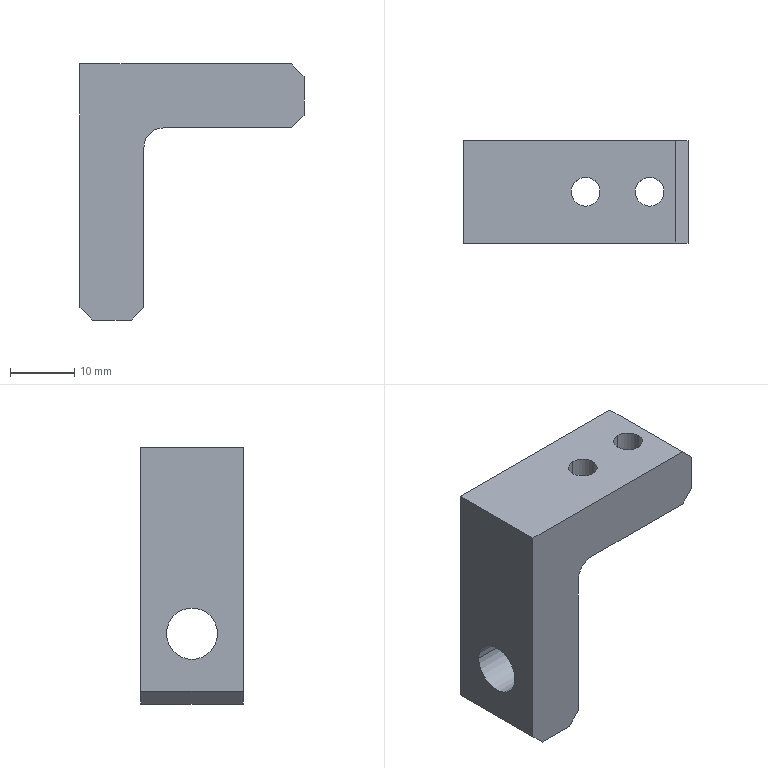Component | SolidWorks | CCDJSStopBlock01-1 | 1 solid | 25 faces | box 35 x 16 x 40 mm | volume 9180 mm3 | plane 14 | cylinder 11 | commonest cylinder face diameters 8 x6 4.5 x4 6 x1 | material 45#
build123d program:
from build123d import *

# Parameters (mm, degrees)
BOSS_EXTRUDE1_DEPTH                             = 16
FILLET1_R                                       = 3
CHAMFER1_SIZE                                   = 2
M8X1_0_TAPPED_HOLE1_D                           = 8
M4_HEX_SOCKET_HEAD_CAP_SCREW_CBORE1_D           = 4.5
M4_HEX_SOCKET_HEAD_CAP_SCREW_CBORE1_CBORE_D     = 8
M4_HEX_SOCKET_HEAD_CAP_SCREW_CBORE1_CBORE_DEPTH = 4.4


with BuildPart() as part:
    # Sketch1 → Boss-Extrude1 (new body)
    with BuildSketch(Plane.XY):
        Polygon((0, 0), (25, 0), (25, -10), (-10, -10), (-10, 30), (0, 30), align=None)
    extrude(amount=BOSS_EXTRUDE1_DEPTH)

    # Fillet1
    fillet1_edges = [part.edges().sort_by_distance(p)[0] for p in [
        (0, 0, 8),
    ]]
    fillet(fillet1_edges, radius=FILLET1_R)

    # Chamfer1
    chamfer1_edges = [part.edges().sort_by_distance(p)[0] for p in [
        (25, 0, 8),
        (25, -10, 8),
        (-10, 30, 8),
        (0, 30, 8),
    ]]
    chamfer(chamfer1_edges, length=CHAMFER1_SIZE)

    # M8x1.0 Tapped Hole1 (through all)
    with Locations(Plane.ZY.offset(10)):
        with Locations((8, 19)):
            Hole(M8X1_0_TAPPED_HOLE1_D / 2)

    # M4 Hex Socket Head Cap Screw CBORE1 (through all)
    with Locations(Plane(origin=(0, 0, 0), x_dir=(1, 0, 0), z_dir=(0, 1, 0))):
        with Locations((19, -8), (9, -8)):
            CounterBoreHole(M4_HEX_SOCKET_HEAD_CAP_SCREW_CBORE1_D / 2, M4_HEX_SOCKET_HEAD_CAP_SCREW_CBORE1_CBORE_D / 2, M4_HEX_SOCKET_HEAD_CAP_SCREW_CBORE1_CBORE_DEPTH)


solid = part.part

# Placed as in the assembly
solid = solid.moved(Location((-208, 391.564, -44.5), (-90, 0, 0)))
STEP:
#1=COLOUR_RGB('',0.7922,0.8196,0.9333);
#2=FILL_AREA_STYLE_COLOUR('',#1);
#3=FILL_AREA_STYLE('',(#2));
#4=SURFACE_STYLE_FILL_AREA(#3);
#5=SURFACE_SIDE_STYLE('',(#4));
#6=SURFACE_STYLE_USAGE(.BOTH.,#5);
#7=PRESENTATION_STYLE_ASSIGNMENT((#6));
#8=CARTESIAN_POINT('',(-7.835,15.573,-1.579));
#9=VERTEX_POINT('',#8);
#10=CARTESIAN_POINT('',(-7.835,15.888,-1.579));
#11=VERTEX_POINT('',#10);
#12=CARTESIAN_POINT('',(-7.835,15.731,-1.579));
#13=DIRECTION('',(-0.,0.,-1.));
#14=DIRECTION('',(0.,1.,0.));
#15=AXIS2_PLACEMENT_3D('',#12,#13,#14);
#16=CIRCLE('',#15,0.1575);
#17=EDGE_CURVE('',#9,#11,#16,.T.);
#18=ORIENTED_EDGE('',*,*,#17,.F.);
#19=CARTESIAN_POINT('',(-7.835,15.573,-1.752));
#20=VERTEX_POINT('',#19);
#21=CARTESIAN_POINT('',(-7.835,15.573,-1.752));
#22=DIRECTION('',(-0.,0.,-1.));
#23=VECTOR('',#22,39.37);
#24=LINE('',#21,#23);
#25=EDGE_CURVE('',#9,#20,#24,.T.);
#26=ORIENTED_EDGE('',*,*,#25,.T.);
#27=CARTESIAN_POINT('',(-7.835,15.888,-1.752));
#28=VERTEX_POINT('',#27);
#29=CARTESIAN_POINT('',(-7.835,15.731,-1.752));
#30=DIRECTION('',(-0.,0.,-1.));
#31=DIRECTION('',(0.,1.,0.));
#32=AXIS2_PLACEMENT_3D('',#29,#30,#31);
#33=CIRCLE('',#32,0.1575);
#34=EDGE_CURVE('',#20,#28,#33,.T.);
#35=ORIENTED_EDGE('',*,*,#34,.T.);
#36=CARTESIAN_POINT('',(-7.835,15.888,-1.752));
#37=DIRECTION('',(-0.,0.,-1.));
#38=VECTOR('',#37,39.37);
#39=LINE('',#36,#38);
#40=EDGE_CURVE('',#11,#28,#39,.T.);
#41=ORIENTED_EDGE('',*,*,#40,.F.);
#42=EDGE_LOOP('',(#18,#26,#35,#41));
#43=FACE_OUTER_BOUND('',#42,.T.);
#44=CARTESIAN_POINT('',(-7.835,15.731,-1.752));
#45=DIRECTION('',(-0.,0.,-1.));
#46=DIRECTION('',(0.,1.,0.));
#47=AXIS2_PLACEMENT_3D('',#44,#45,#46);
#48=CYLINDRICAL_SURFACE('',#47,0.1575);
#49=ADVANCED_FACE('',(#43),#48,.F.);
#50=CARTESIAN_POINT('',(-7.835,15.642,-1.358));
#51=VERTEX_POINT('',#50);
#52=CARTESIAN_POINT('',(-7.835,15.819,-1.358));
#53=VERTEX_POINT('',#52);
#54=CARTESIAN_POINT('',(-7.835,15.731,-1.358));
#55=DIRECTION('',(-0.,0.,-1.));
#56=DIRECTION('',(0.,1.,0.));
#57=AXIS2_PLACEMENT_3D('',#54,#55,#56);
#58=CIRCLE('',#57,0.08858);
#59=EDGE_CURVE('',#51,#53,#58,.T.);
#60=ORIENTED_EDGE('',*,*,#59,.F.);
#61=CARTESIAN_POINT('',(-7.835,15.642,-1.579));
#62=VERTEX_POINT('',#61);
#63=CARTESIAN_POINT('',(-7.835,15.642,-1.752));
#64=DIRECTION('',(-0.,0.,-1.));
#65=VECTOR('',#64,39.37);
#66=LINE('',#63,#65);
#67=EDGE_CURVE('',#51,#62,#66,.T.);
#68=ORIENTED_EDGE('',*,*,#67,.T.);
#69=CARTESIAN_POINT('',(-7.835,15.819,-1.579));
#70=VERTEX_POINT('',#69);
#71=CARTESIAN_POINT('',(-7.835,15.731,-1.579));
#72=DIRECTION('',(-0.,0.,-1.));
#73=DIRECTION('',(0.,1.,0.));
#74=AXIS2_PLACEMENT_3D('',#71,#72,#73);
#75=CIRCLE('',#74,0.08858);
#76=EDGE_CURVE('',#62,#70,#75,.T.);
#77=ORIENTED_EDGE('',*,*,#76,.T.);
#78=CARTESIAN_POINT('',(-7.835,15.819,-1.752));
#79=DIRECTION('',(-0.,0.,-1.));
#80=VECTOR('',#79,39.37);
#81=LINE('',#78,#80);
#82=EDGE_CURVE('',#53,#70,#81,.T.);
#83=ORIENTED_EDGE('',*,*,#82,.F.);
#84=EDGE_LOOP('',(#60,#68,#77,#83));
#85=FACE_OUTER_BOUND('',#84,.T.);
#86=CARTESIAN_POINT('',(-7.835,15.731,-1.752));
#87=DIRECTION('',(-0.,0.,-1.));
#88=DIRECTION('',(0.,1.,0.));
#89=AXIS2_PLACEMENT_3D('',#86,#87,#88);
#90=CYLINDRICAL_SURFACE('',#89,0.08858);
#91=ADVANCED_FACE('',(#85),#90,.F.);
#92=CARTESIAN_POINT('',(-7.441,15.573,-1.579));
#93=VERTEX_POINT('',#92);
#94=CARTESIAN_POINT('',(-7.441,15.888,-1.579));
#95=VERTEX_POINT('',#94);
#96=CARTESIAN_POINT('',(-7.441,15.731,-1.579));
#97=DIRECTION('',(-0.,0.,-1.));
#98=DIRECTION('',(0.,1.,0.));
#99=AXIS2_PLACEMENT_3D('',#96,#97,#98);
#100=CIRCLE('',#99,0.1575);
#101=EDGE_CURVE('',#93,#95,#100,.T.);
#102=ORIENTED_EDGE('',*,*,#101,.F.);
#103=CARTESIAN_POINT('',(-7.441,15.573,-1.752));
#104=VERTEX_POINT('',#103);
#105=CARTESIAN_POINT('',(-7.441,15.573,-1.752));
#106=DIRECTION('',(-0.,0.,-1.));
#107=VECTOR('',#106,39.37);
#108=LINE('',#105,#107);
#109=EDGE_CURVE('',#93,#104,#108,.T.);
#110=ORIENTED_EDGE('',*,*,#109,.T.);
#111=CARTESIAN_POINT('',(-7.441,15.888,-1.752));
#112=VERTEX_POINT('',#111);
#113=CARTESIAN_POINT('',(-7.441,15.731,-1.752));
#114=DIRECTION('',(-0.,0.,-1.));
#115=DIRECTION('',(0.,1.,0.));
#116=AXIS2_PLACEMENT_3D('',#113,#114,#115);
#117=CIRCLE('',#116,0.1575);
#118=EDGE_CURVE('',#104,#112,#117,.T.);
#119=ORIENTED_EDGE('',*,*,#118,.T.);
#120=CARTESIAN_POINT('',(-7.441,15.888,-1.752));
#121=DIRECTION('',(-0.,0.,-1.));
#122=VECTOR('',#121,39.37);
#123=LINE('',#120,#122);
#124=EDGE_CURVE('',#95,#112,#123,.T.);
#125=ORIENTED_EDGE('',*,*,#124,.F.);
#126=EDGE_LOOP('',(#102,#110,#119,#125));
#127=FACE_OUTER_BOUND('',#126,.T.);
#128=CARTESIAN_POINT('',(-7.441,15.731,-1.752));
#129=DIRECTION('',(-0.,0.,-1.));
#130=DIRECTION('',(0.,1.,0.));
#131=AXIS2_PLACEMENT_3D('',#128,#129,#130);
#132=CYLINDRICAL_SURFACE('',#131,0.1575);
#133=ADVANCED_FACE('',(#127),#132,.F.);
#134=CARTESIAN_POINT('',(-7.441,15.642,-1.358));
#135=VERTEX_POINT('',#134);
#136=CARTESIAN_POINT('',(-7.441,15.819,-1.358));
#137=VERTEX_POINT('',#136);
#138=CARTESIAN_POINT('',(-7.441,15.731,-1.358));
#139=DIRECTION('',(-0.,0.,-1.));
#140=DIRECTION('',(0.,1.,0.));
#141=AXIS2_PLACEMENT_3D('',#138,#139,#140);
#142=CIRCLE('',#141,0.08858);
#143=EDGE_CURVE('',#135,#137,#142,.T.);
#144=ORIENTED_EDGE('',*,*,#143,.F.);
#145=CARTESIAN_POINT('',(-7.441,15.642,-1.579));
#146=VERTEX_POINT('',#145);
#147=CARTESIAN_POINT('',(-7.441,15.642,-1.752));
#148=DIRECTION('',(-0.,0.,-1.));
#149=VECTOR('',#148,39.37);
#150=LINE('',#147,#149);
#151=EDGE_CURVE('',#135,#146,#150,.T.);
#152=ORIENTED_EDGE('',*,*,#151,.T.);
#153=CARTESIAN_POINT('',(-7.441,15.819,-1.579));
#154=VERTEX_POINT('',#153);
#155=CARTESIAN_POINT('',(-7.441,15.731,-1.579));
#156=DIRECTION('',(-0.,0.,-1.));
#157=DIRECTION('',(0.,1.,0.));
#158=AXIS2_PLACEMENT_3D('',#155,#156,#157);
#159=CIRCLE('',#158,0.08858);
#160=EDGE_CURVE('',#146,#154,#159,.T.);
#161=ORIENTED_EDGE('',*,*,#160,.T.);
#162=CARTESIAN_POINT('',(-7.441,15.819,-1.752));
#163=DIRECTION('',(-0.,0.,-1.));
#164=VECTOR('',#163,39.37);
#165=LINE('',#162,#164);
#166=EDGE_CURVE('',#137,#154,#165,.T.);
#167=ORIENTED_EDGE('',*,*,#166,.F.);
#168=EDGE_LOOP('',(#144,#152,#161,#167));
#169=FACE_OUTER_BOUND('',#168,.T.);
#170=CARTESIAN_POINT('',(-7.441,15.731,-1.752));
#171=DIRECTION('',(-0.,0.,-1.));
#172=DIRECTION('',(0.,1.,0.));
#173=AXIS2_PLACEMENT_3D('',#170,#171,#172);
#174=CYLINDRICAL_SURFACE('',#173,0.08858);
#175=ADVANCED_FACE('',(#169),#174,.F.);
#176=CARTESIAN_POINT('',(-8.189,15.573,-2.5));
#177=VERTEX_POINT('',#176);
#178=CARTESIAN_POINT('',(-8.189,15.888,-2.5));
#179=VERTEX_POINT('',#178);
#180=CARTESIAN_POINT('',(-8.189,15.731,-2.5));
#181=DIRECTION('',(-1.,0.,-0.));
#182=DIRECTION('',(0.,0.,1.));
#183=AXIS2_PLACEMENT_3D('',#180,#181,#182);
#184=CIRCLE('',#183,0.1575);
#185=EDGE_CURVE('',#177,#179,#184,.T.);
#186=ORIENTED_EDGE('',*,*,#185,.F.);
#187=CARTESIAN_POINT('',(-8.583,15.573,-2.5));
#188=VERTEX_POINT('',#187);
#189=CARTESIAN_POINT('',(-8.583,15.573,-2.5));
#190=DIRECTION('',(-1.,0.,0.));
#191=VECTOR('',#190,39.37);
#192=LINE('',#189,#191);
#193=EDGE_CURVE('',#177,#188,#192,.T.);
#194=ORIENTED_EDGE('',*,*,#193,.T.);
#195=CARTESIAN_POINT('',(-8.583,15.888,-2.5));
#196=VERTEX_POINT('',#195);
#197=CARTESIAN_POINT('',(-8.583,15.731,-2.5));
#198=DIRECTION('',(-1.,0.,0.));
#199=DIRECTION('',(0.,1.,0.));
#200=AXIS2_PLACEMENT_3D('',#197,#198,#199);
#201=CIRCLE('',#200,0.1575);
#202=EDGE_CURVE('',#188,#196,#201,.T.);
#203=ORIENTED_EDGE('',*,*,#202,.T.);
#204=CARTESIAN_POINT('',(-8.583,15.888,-2.5));
#205=DIRECTION('',(-1.,0.,0.));
#206=VECTOR('',#205,39.37);
#207=LINE('',#204,#206);
#208=EDGE_CURVE('',#179,#196,#207,.T.);
#209=ORIENTED_EDGE('',*,*,#208,.F.);
#210=EDGE_LOOP('',(#186,#194,#203,#209));
#211=FACE_OUTER_BOUND('',#210,.T.);
#212=CARTESIAN_POINT('',(-8.583,15.731,-2.5));
#213=DIRECTION('',(-1.,0.,0.));
#214=DIRECTION('',(0.,1.,0.));
#215=AXIS2_PLACEMENT_3D('',#212,#213,#214);
#216=CYLINDRICAL_SURFACE('',#215,0.1575);
#217=ADVANCED_FACE('',(#211),#216,.F.);
#218=CARTESIAN_POINT('',(-8.189,15.731,-2.5));
#219=DIRECTION('',(-1.,0.,-0.));
#220=DIRECTION('',(0.,0.,1.));
#221=AXIS2_PLACEMENT_3D('',#218,#219,#220);
#222=CIRCLE('',#221,0.1575);
#223=EDGE_CURVE('',#179,#177,#222,.T.);
#224=ORIENTED_EDGE('',*,*,#223,.T.);
#225=ORIENTED_EDGE('',*,*,#185,.T.);
#226=EDGE_LOOP('',(#224,#225));
#227=FACE_BOUND('',#226,.T.);
#228=CARTESIAN_POINT('',(-8.189,15.416,-1.87));
#229=VERTEX_POINT('',#228);
#230=CARTESIAN_POINT('',(-8.189,15.416,-2.854));
#231=VERTEX_POINT('',#230);
#232=CARTESIAN_POINT('',(-8.189,15.416,-2.933));
#233=DIRECTION('',(0.,0.,-1.));
#234=VECTOR('',#233,39.37);
#235=LINE('',#232,#234);
#236=EDGE_CURVE('',#229,#231,#235,.T.);
#237=ORIENTED_EDGE('',*,*,#236,.T.);
#238=CARTESIAN_POINT('',(-8.189,16.046,-2.854));
#239=VERTEX_POINT('',#238);
#240=CARTESIAN_POINT('',(-8.189,16.046,-2.854));
#241=DIRECTION('',(0.,1.,0.));
#242=VECTOR('',#241,39.37);
#243=LINE('',#240,#242);
#244=EDGE_CURVE('',#231,#239,#243,.T.);
#245=ORIENTED_EDGE('',*,*,#244,.T.);
#246=CARTESIAN_POINT('',(-8.189,16.046,-1.87));
#247=VERTEX_POINT('',#246);
#248=CARTESIAN_POINT('',(-8.189,16.046,-2.933));
#249=DIRECTION('',(0.,0.,-1.));
#250=VECTOR('',#249,39.37);
#251=LINE('',#248,#250);
#252=EDGE_CURVE('',#247,#239,#251,.T.);
#253=ORIENTED_EDGE('',*,*,#252,.F.);
#254=CARTESIAN_POINT('',(-8.189,15.416,-1.87));
#255=DIRECTION('',(-0.,-1.,-0.));
#256=VECTOR('',#255,39.37);
#257=LINE('',#254,#256);
#258=EDGE_CURVE('',#247,#229,#257,.T.);
#259=ORIENTED_EDGE('',*,*,#258,.T.);
#260=EDGE_LOOP('',(#237,#245,#253,#259));
#261=FACE_OUTER_BOUND('',#260,.T.);
#262=CARTESIAN_POINT('',(-8.189,16.046,-2.933));
#263=DIRECTION('',(-1.,0.,-0.));
#264=DIRECTION('',(-0.,-0.,1.));
#265=AXIS2_PLACEMENT_3D('',#262,#263,#264);
#266=PLANE('',#265);
#267=ADVANCED_FACE('',(#227,#261),#266,.F.);
#268=CARTESIAN_POINT('',(-8.268,15.416,-2.933));
#269=VERTEX_POINT('',#268);
#270=CARTESIAN_POINT('',(-8.504,15.416,-2.933));
#271=VERTEX_POINT('',#270);
#272=CARTESIAN_POINT('',(-8.583,15.416,-2.933));
#273=DIRECTION('',(-1.,0.,0.));
#274=VECTOR('',#273,39.37);
#275=LINE('',#272,#274);
#276=EDGE_CURVE('',#269,#271,#275,.T.);
#277=ORIENTED_EDGE('',*,*,#276,.T.);
#278=CARTESIAN_POINT('',(-8.504,16.046,-2.933));
#279=VERTEX_POINT('',#278);
#280=CARTESIAN_POINT('',(-8.504,16.046,-2.933));
#281=DIRECTION('',(0.,1.,0.));
#282=VECTOR('',#281,39.37);
#283=LINE('',#280,#282);
#284=EDGE_CURVE('',#271,#279,#283,.T.);
#285=ORIENTED_EDGE('',*,*,#284,.T.);
#286=CARTESIAN_POINT('',(-8.268,16.046,-2.933));
#287=VERTEX_POINT('',#286);
#288=CARTESIAN_POINT('',(-8.583,16.046,-2.933));
#289=DIRECTION('',(-1.,0.,0.));
#290=VECTOR('',#289,39.37);
#291=LINE('',#288,#290);
#292=EDGE_CURVE('',#287,#279,#291,.T.);
#293=ORIENTED_EDGE('',*,*,#292,.F.);
#294=CARTESIAN_POINT('',(-8.268,16.046,-2.933));
#295=DIRECTION('',(-0.,-1.,-0.));
#296=VECTOR('',#295,39.37);
#297=LINE('',#294,#296);
#298=EDGE_CURVE('',#287,#269,#297,.T.);
#299=ORIENTED_EDGE('',*,*,#298,.T.);
#300=EDGE_LOOP('',(#277,#285,#293,#299));
#301=FACE_OUTER_BOUND('',#300,.T.);
#302=CARTESIAN_POINT('',(-8.583,16.046,-2.933));
#303=DIRECTION('',(0.,-0.,1.));
#304=DIRECTION('',(-0.,-1.,-0.));
#305=AXIS2_PLACEMENT_3D('',#302,#303,#304);
#306=PLANE('',#305);
#307=ADVANCED_FACE('',(#301),#306,.F.);
#308=CARTESIAN_POINT('',(-8.583,15.731,-2.5));
#309=DIRECTION('',(-1.,0.,0.));
#310=DIRECTION('',(0.,1.,0.));
#311=AXIS2_PLACEMENT_3D('',#308,#309,#310);
#312=CIRCLE('',#311,0.1575);
#313=EDGE_CURVE('',#196,#188,#312,.T.);
#314=ORIENTED_EDGE('',*,*,#313,.F.);
#315=ORIENTED_EDGE('',*,*,#202,.F.);
#316=EDGE_LOOP('',(#314,#315));
#317=FACE_BOUND('',#316,.T.);
#318=CARTESIAN_POINT('',(-8.583,16.046,-2.854));
#319=VERTEX_POINT('',#318);
#320=CARTESIAN_POINT('',(-8.583,16.046,-1.358));
#321=VERTEX_POINT('',#320);
#322=CARTESIAN_POINT('',(-8.583,16.046,-1.358));
#323=DIRECTION('',(0.,-0.,1.));
#324=VECTOR('',#323,39.37);
#325=LINE('',#322,#324);
#326=EDGE_CURVE('',#319,#321,#325,.T.);
#327=ORIENTED_EDGE('',*,*,#326,.F.);
#328=CARTESIAN_POINT('',(-8.583,15.416,-2.854));
#329=VERTEX_POINT('',#328);
#330=CARTESIAN_POINT('',(-8.583,16.046,-2.854));
#331=DIRECTION('',(-0.,-1.,-0.));
#332=VECTOR('',#331,39.37);
#333=LINE('',#330,#332);
#334=EDGE_CURVE('',#319,#329,#333,.T.);
#335=ORIENTED_EDGE('',*,*,#334,.T.);
#336=CARTESIAN_POINT('',(-8.583,15.416,-1.358));
#337=VERTEX_POINT('',#336);
#338=CARTESIAN_POINT('',(-8.583,15.416,-1.358));
#339=DIRECTION('',(0.,-0.,1.));
#340=VECTOR('',#339,39.37);
#341=LINE('',#338,#340);
#342=EDGE_CURVE('',#329,#337,#341,.T.);
#343=ORIENTED_EDGE('',*,*,#342,.T.);
#344=CARTESIAN_POINT('',(-8.583,16.046,-1.358));
#345=DIRECTION('',(-0.,-1.,-0.));
#346=VECTOR('',#345,39.37);
#347=LINE('',#344,#346);
#348=EDGE_CURVE('',#321,#337,#347,.T.);
#349=ORIENTED_EDGE('',*,*,#348,.F.);
#350=EDGE_LOOP('',(#327,#335,#343,#349));
#351=FACE_OUTER_BOUND('',#350,.T.);
#352=CARTESIAN_POINT('',(-8.583,16.046,-1.358));
#353=DIRECTION('',(1.,-0.,-0.));
#354=DIRECTION('',(-0.,-1.,-0.));
#355=AXIS2_PLACEMENT_3D('',#352,#353,#354);
#356=PLANE('',#355);
#357=ADVANCED_FACE('',(#317,#351),#356,.F.);
#358=CARTESIAN_POINT('',(-7.835,15.731,-1.358));
#359=DIRECTION('',(-0.,0.,-1.));
#360=DIRECTION('',(0.,1.,0.));
#361=AXIS2_PLACEMENT_3D('',#358,#359,#360);
#362=CIRCLE('',#361,0.08858);
#363=EDGE_CURVE('',#53,#51,#362,.T.);
#364=ORIENTED_EDGE('',*,*,#363,.T.);
#365=ORIENTED_EDGE('',*,*,#59,.T.);
#366=EDGE_LOOP('',(#364,#365));
#367=FACE_BOUND('',#366,.T.);
#368=CARTESIAN_POINT('',(-7.441,15.731,-1.358));
#369=DIRECTION('',(-0.,0.,-1.));
#370=DIRECTION('',(0.,1.,0.));
#371=AXIS2_PLACEMENT_3D('',#368,#369,#370);
#372=CIRCLE('',#371,0.08858);
#373=EDGE_CURVE('',#137,#135,#372,.T.);
#374=ORIENTED_EDGE('',*,*,#373,.T.);
#375=ORIENTED_EDGE('',*,*,#143,.T.);
#376=EDGE_LOOP('',(#374,#375));
#377=FACE_BOUND('',#376,.T.);
#378=CARTESIAN_POINT('',(-7.283,15.416,-1.358));
#379=VERTEX_POINT('',#378);
#380=CARTESIAN_POINT('',(-7.205,15.416,-1.358));
#381=DIRECTION('',(1.,-0.,-0.));
#382=VECTOR('',#381,39.37);
#383=LINE('',#380,#382);
#384=EDGE_CURVE('',#337,#379,#383,.T.);
#385=ORIENTED_EDGE('',*,*,#384,.T.);
#386=CARTESIAN_POINT('',(-7.283,16.046,-1.358));
#387=VERTEX_POINT('',#386);
#388=CARTESIAN_POINT('',(-7.283,16.046,-1.358));
#389=DIRECTION('',(0.,1.,0.));
#390=VECTOR('',#389,39.37);
#391=LINE('',#388,#390);
#392=EDGE_CURVE('',#379,#387,#391,.T.);
#393=ORIENTED_EDGE('',*,*,#392,.T.);
#394=CARTESIAN_POINT('',(-7.205,16.046,-1.358));
#395=DIRECTION('',(1.,-0.,-0.));
#396=VECTOR('',#395,39.37);
#397=LINE('',#394,#396);
#398=EDGE_CURVE('',#321,#387,#397,.T.);
#399=ORIENTED_EDGE('',*,*,#398,.F.);
#400=ORIENTED_EDGE('',*,*,#348,.T.);
#401=EDGE_LOOP('',(#385,#393,#399,#400));
#402=FACE_OUTER_BOUND('',#401,.T.);
#403=CARTESIAN_POINT('',(-7.205,16.046,-1.358));
#404=DIRECTION('',(-0.,0.,-1.));
#405=DIRECTION('',(-1.,0.,0.));
#406=AXIS2_PLACEMENT_3D('',#403,#404,#405);
#407=PLANE('',#406);
#408=ADVANCED_FACE('',(#367,#377,#402),#407,.F.);
#409=CARTESIAN_POINT('',(-7.205,16.046,-1.437));
#410=VERTEX_POINT('',#409);
#411=CARTESIAN_POINT('',(-7.205,16.046,-1.673));
#412=VERTEX_POINT('',#411);
#413=CARTESIAN_POINT('',(-7.205,16.046,-1.752));
#414=DIRECTION('',(-0.,0.,-1.));
#415=VECTOR('',#414,39.37);
#416=LINE('',#413,#415);
#417=EDGE_CURVE('',#410,#412,#416,.T.);
#418=ORIENTED_EDGE('',*,*,#417,.F.);
#419=CARTESIAN_POINT('',(-7.205,15.416,-1.437));
#420=VERTEX_POINT('',#419);
#421=CARTESIAN_POINT('',(-7.205,16.046,-1.437));
#422=DIRECTION('',(-0.,-1.,-0.));
#423=VECTOR('',#422,39.37);
#424=LINE('',#421,#423);
#425=EDGE_CURVE('',#410,#420,#424,.T.);
#426=ORIENTED_EDGE('',*,*,#425,.T.);
#427=CARTESIAN_POINT('',(-7.205,15.416,-1.673));
#428=VERTEX_POINT('',#427);
#429=CARTESIAN_POINT('',(-7.205,15.416,-1.752));
#430=DIRECTION('',(-0.,0.,-1.));
#431=VECTOR('',#430,39.37);
#432=LINE('',#429,#431);
#433=EDGE_CURVE('',#420,#428,#432,.T.);
#434=ORIENTED_EDGE('',*,*,#433,.T.);
#435=CARTESIAN_POINT('',(-7.205,16.046,-1.673));
#436=DIRECTION('',(0.,1.,0.));
#437=VECTOR('',#436,39.37);
#438=LINE('',#435,#437);
#439=EDGE_CURVE('',#428,#412,#438,.T.);
#440=ORIENTED_EDGE('',*,*,#439,.T.);
#441=EDGE_LOOP('',(#418,#426,#434,#440));
#442=FACE_OUTER_BOUND('',#441,.T.);
#443=CARTESIAN_POINT('',(-7.205,16.046,-1.752));
#444=DIRECTION('',(-1.,0.,0.));
#445=DIRECTION('',(0.,1.,0.));
#446=AXIS2_PLACEMENT_3D('',#443,#444,#445);
#447=PLANE('',#446);
#448=ADVANCED_FACE('',(#442),#447,.F.);
#449=CARTESIAN_POINT('',(-7.835,15.731,-1.752));
#450=DIRECTION('',(-0.,0.,-1.));
#451=DIRECTION('',(0.,1.,0.));
#452=AXIS2_PLACEMENT_3D('',#449,#450,#451);
#453=CIRCLE('',#452,0.1575);
#454=EDGE_CURVE('',#28,#20,#453,.T.);
#455=ORIENTED_EDGE('',*,*,#454,.F.);
#456=ORIENTED_EDGE('',*,*,#34,.F.);
#457=EDGE_LOOP('',(#455,#456));
#458=FACE_BOUND('',#457,.T.);
#459=CARTESIAN_POINT('',(-7.283,16.046,-1.752));
#460=VERTEX_POINT('',#459);
#461=CARTESIAN_POINT('',(-7.283,15.731,-1.752));
#462=VERTEX_POINT('',#461);
#463=CARTESIAN_POINT('',(-7.283,16.046,-1.752));
#464=DIRECTION('',(-0.,-1.,-0.));
#465=VECTOR('',#464,39.37);
#466=LINE('',#463,#465);
#467=EDGE_CURVE('',#460,#462,#466,.T.);
#468=ORIENTED_EDGE('',*,*,#467,.T.);
#469=CARTESIAN_POINT('',(-7.441,15.731,-1.752));
#470=DIRECTION('',(-0.,0.,-1.));
#471=DIRECTION('',(0.,1.,0.));
#472=AXIS2_PLACEMENT_3D('',#469,#470,#471);
#473=CIRCLE('',#472,0.1575);
#474=EDGE_CURVE('',#112,#462,#473,.T.);
#475=ORIENTED_EDGE('',*,*,#474,.F.);
#476=ORIENTED_EDGE('',*,*,#118,.F.);
#477=CARTESIAN_POINT('',(-7.441,15.731,-1.752));
#478=DIRECTION('',(-0.,0.,-1.));
#479=DIRECTION('',(0.,1.,0.));
#480=AXIS2_PLACEMENT_3D('',#477,#478,#479);
#481=CIRCLE('',#480,0.1575);
#482=EDGE_CURVE('',#462,#104,#481,.T.);
#483=ORIENTED_EDGE('',*,*,#482,.F.);
#484=CARTESIAN_POINT('',(-7.283,15.416,-1.752));
#485=VERTEX_POINT('',#484);
#486=CARTESIAN_POINT('',(-7.283,16.046,-1.752));
#487=DIRECTION('',(-0.,-1.,-0.));
#488=VECTOR('',#487,39.37);
#489=LINE('',#486,#488);
#490=EDGE_CURVE('',#462,#485,#489,.T.);
#491=ORIENTED_EDGE('',*,*,#490,.T.);
#492=CARTESIAN_POINT('',(-8.071,15.416,-1.752));
#493=VERTEX_POINT('',#492);
#494=CARTESIAN_POINT('',(-8.189,15.416,-1.752));
#495=DIRECTION('',(-1.,0.,0.));
#496=VECTOR('',#495,39.37);
#497=LINE('',#494,#496);
#498=EDGE_CURVE('',#485,#493,#497,.T.);
#499=ORIENTED_EDGE('',*,*,#498,.T.);
#500=CARTESIAN_POINT('',(-8.071,16.046,-1.752));
#501=VERTEX_POINT('',#500);
#502=CARTESIAN_POINT('',(-8.071,16.046,-1.752));
#503=DIRECTION('',(0.,1.,0.));
#504=VECTOR('',#503,39.37);
#505=LINE('',#502,#504);
#506=EDGE_CURVE('',#493,#501,#505,.T.);
#507=ORIENTED_EDGE('',*,*,#506,.T.);
#508=CARTESIAN_POINT('',(-8.189,16.046,-1.752));
#509=DIRECTION('',(-1.,0.,0.));
#510=VECTOR('',#509,39.37);
#511=LINE('',#508,#510);
#512=EDGE_CURVE('',#460,#501,#511,.T.);
#513=ORIENTED_EDGE('',*,*,#512,.F.);
#514=EDGE_LOOP('',(#468,#475,#476,#483,#491,#499,#507,#513));
#515=FACE_OUTER_BOUND('',#514,.T.);
#516=CARTESIAN_POINT('',(-8.189,16.046,-1.752));
#517=DIRECTION('',(0.,-0.,1.));
#518=DIRECTION('',(-0.,-1.,-0.));
#519=AXIS2_PLACEMENT_3D('',#516,#517,#518);
#520=PLANE('',#519);
#521=ADVANCED_FACE('',(#458,#515),#520,.F.);
#522=ORIENTED_EDGE('',*,*,#398,.T.);
#523=CARTESIAN_POINT('',(-7.539,16.046,-1.102));
#524=DIRECTION('',(0.7071,-0.,-0.7071));
#525=VECTOR('',#524,39.37);
#526=LINE('',#523,#525);
#527=EDGE_CURVE('',#387,#410,#526,.T.);
#528=ORIENTED_EDGE('',*,*,#527,.T.);
#529=ORIENTED_EDGE('',*,*,#417,.T.);
#530=CARTESIAN_POINT('',(-7.736,16.046,-2.205));
#531=DIRECTION('',(-0.7071,0.,-0.7071));
#532=VECTOR('',#531,39.37);
#533=LINE('',#530,#532);
#534=EDGE_CURVE('',#412,#460,#533,.T.);
#535=ORIENTED_EDGE('',*,*,#534,.T.);
#536=ORIENTED_EDGE('',*,*,#512,.T.);
#537=CARTESIAN_POINT('',(-8.071,16.046,-1.87));
#538=DIRECTION('',(-0.,-1.,-0.));
#539=DIRECTION('',(1.,0.,0.));
#540=AXIS2_PLACEMENT_3D('',#537,#538,#539);
#541=CIRCLE('',#540,0.1181);
#542=EDGE_CURVE('',#501,#247,#541,.T.);
#543=ORIENTED_EDGE('',*,*,#542,.T.);
#544=ORIENTED_EDGE('',*,*,#252,.T.);
#545=CARTESIAN_POINT('',(-7.638,16.046,-2.303));
#546=DIRECTION('',(-0.7071,0.,-0.7071));
#547=VECTOR('',#546,39.37);
#548=LINE('',#545,#547);
#549=EDGE_CURVE('',#239,#287,#548,.T.);
#550=ORIENTED_EDGE('',*,*,#549,.T.);
#551=ORIENTED_EDGE('',*,*,#292,.T.);
#552=CARTESIAN_POINT('',(-8.937,16.046,-2.5));
#553=DIRECTION('',(-0.7071,0.,0.7071));
#554=VECTOR('',#553,39.37);
#555=LINE('',#552,#554);
#556=EDGE_CURVE('',#279,#319,#555,.T.);
#557=ORIENTED_EDGE('',*,*,#556,.T.);
#558=ORIENTED_EDGE('',*,*,#326,.T.);
#559=EDGE_LOOP('',(#522,#528,#529,#535,#536,#543,#544,#550,#551,#557,#558));
#560=FACE_OUTER_BOUND('',#559,.T.);
#561=CARTESIAN_POINT('',(-8.189,16.046,-1.752));
#562=DIRECTION('',(0.,1.,0.));
#563=DIRECTION('',(1.,-0.,-0.));
#564=AXIS2_PLACEMENT_3D('',#561,#562,#563);
#565=PLANE('',#564);
#566=ADVANCED_FACE('',(#560),#565,.T.);
#567=ORIENTED_EDGE('',*,*,#433,.F.);
#568=CARTESIAN_POINT('',(-7.205,15.416,-1.437));
#569=DIRECTION('',(-0.7071,0.,0.7071));
#570=VECTOR('',#569,39.37);
#571=LINE('',#568,#570);
#572=EDGE_CURVE('',#420,#379,#571,.T.);
#573=ORIENTED_EDGE('',*,*,#572,.T.);
#574=ORIENTED_EDGE('',*,*,#384,.F.);
#575=ORIENTED_EDGE('',*,*,#342,.F.);
#576=CARTESIAN_POINT('',(-8.583,15.416,-2.854));
#577=DIRECTION('',(0.7071,-0.,-0.7071));
#578=VECTOR('',#577,39.37);
#579=LINE('',#576,#578);
#580=EDGE_CURVE('',#329,#271,#579,.T.);
#581=ORIENTED_EDGE('',*,*,#580,.T.);
#582=ORIENTED_EDGE('',*,*,#276,.F.);
#583=CARTESIAN_POINT('',(-8.268,15.416,-2.933));
#584=DIRECTION('',(0.7071,-0.,0.7071));
#585=VECTOR('',#584,39.37);
#586=LINE('',#583,#585);
#587=EDGE_CURVE('',#269,#231,#586,.T.);
#588=ORIENTED_EDGE('',*,*,#587,.T.);
#589=ORIENTED_EDGE('',*,*,#236,.F.);
#590=CARTESIAN_POINT('',(-8.071,15.416,-1.87));
#591=DIRECTION('',(0.,1.,0.));
#592=DIRECTION('',(1.,0.,0.));
#593=AXIS2_PLACEMENT_3D('',#590,#591,#592);
#594=CIRCLE('',#593,0.1181);
#595=EDGE_CURVE('',#229,#493,#594,.T.);
#596=ORIENTED_EDGE('',*,*,#595,.T.);
#597=ORIENTED_EDGE('',*,*,#498,.F.);
#598=CARTESIAN_POINT('',(-7.283,15.416,-1.752));
#599=DIRECTION('',(0.7071,-0.,0.7071));
#600=VECTOR('',#599,39.37);
#601=LINE('',#598,#600);
#602=EDGE_CURVE('',#485,#428,#601,.T.);
#603=ORIENTED_EDGE('',*,*,#602,.T.);
#604=EDGE_LOOP('',(#567,#573,#574,#575,#581,#582,#588,#589,#596,#597,#603));
#605=FACE_OUTER_BOUND('',#604,.T.);
#606=CARTESIAN_POINT('',(-8.189,15.416,-1.752));
#607=DIRECTION('',(0.,1.,0.));
#608=DIRECTION('',(1.,-0.,-0.));
#609=AXIS2_PLACEMENT_3D('',#606,#607,#608);
#610=PLANE('',#609);
#611=ADVANCED_FACE('',(#605),#610,.F.);
#612=ORIENTED_EDGE('',*,*,#542,.F.);
#613=ORIENTED_EDGE('',*,*,#506,.F.);
#614=ORIENTED_EDGE('',*,*,#595,.F.);
#615=ORIENTED_EDGE('',*,*,#258,.F.);
#616=EDGE_LOOP('',(#612,#613,#614,#615));
#617=FACE_OUTER_BOUND('',#616,.T.);
#618=CARTESIAN_POINT('',(-8.071,16.046,-1.87));
#619=DIRECTION('',(0.,1.,0.));
#620=DIRECTION('',(1.,0.,0.));
#621=AXIS2_PLACEMENT_3D('',#618,#619,#620);
#622=CYLINDRICAL_SURFACE('',#621,0.1181);
#623=ADVANCED_FACE('',(#617),#622,.F.);
#624=ORIENTED_EDGE('',*,*,#527,.F.);
#625=ORIENTED_EDGE('',*,*,#392,.F.);
#626=ORIENTED_EDGE('',*,*,#572,.F.);
#627=ORIENTED_EDGE('',*,*,#425,.F.);
#628=EDGE_LOOP('',(#624,#625,#626,#627));
#629=FACE_OUTER_BOUND('',#628,.T.);
#630=CARTESIAN_POINT('',(-7.205,16.046,-1.437));
#631=DIRECTION('',(-0.7071,0.,-0.7071));
#632=DIRECTION('',(-0.,-1.,-0.));
#633=AXIS2_PLACEMENT_3D('',#630,#631,#632);
#634=PLANE('',#633);
#635=ADVANCED_FACE('',(#629),#634,.F.);
#636=ORIENTED_EDGE('',*,*,#534,.F.);
#637=ORIENTED_EDGE('',*,*,#439,.F.);
#638=ORIENTED_EDGE('',*,*,#602,.F.);
#639=ORIENTED_EDGE('',*,*,#490,.F.);
#640=ORIENTED_EDGE('',*,*,#467,.F.);
#641=EDGE_LOOP('',(#636,#637,#638,#639,#640));
#642=FACE_OUTER_BOUND('',#641,.T.);
#643=CARTESIAN_POINT('',(-7.283,16.046,-1.752));
#644=DIRECTION('',(-0.7071,0.,0.7071));
#645=DIRECTION('',(-0.,-1.,-0.));
#646=AXIS2_PLACEMENT_3D('',#643,#644,#645);
#647=PLANE('',#646);
#648=ADVANCED_FACE('',(#642),#647,.F.);
#649=ORIENTED_EDGE('',*,*,#556,.F.);
#650=ORIENTED_EDGE('',*,*,#284,.F.);
#651=ORIENTED_EDGE('',*,*,#580,.F.);
#652=ORIENTED_EDGE('',*,*,#334,.F.);
#653=EDGE_LOOP('',(#649,#650,#651,#652));
#654=FACE_OUTER_BOUND('',#653,.T.);
#655=CARTESIAN_POINT('',(-8.583,16.046,-2.854));
#656=DIRECTION('',(0.7071,-0.,0.7071));
#657=DIRECTION('',(-0.,-1.,-0.));
#658=AXIS2_PLACEMENT_3D('',#655,#656,#657);
#659=PLANE('',#658);
#660=ADVANCED_FACE('',(#654),#659,.F.);
#661=ORIENTED_EDGE('',*,*,#549,.F.);
#662=ORIENTED_EDGE('',*,*,#244,.F.);
#663=ORIENTED_EDGE('',*,*,#587,.F.);
#664=ORIENTED_EDGE('',*,*,#298,.F.);
#665=EDGE_LOOP('',(#661,#662,#663,#664));
#666=FACE_OUTER_BOUND('',#665,.T.);
#667=CARTESIAN_POINT('',(-8.268,16.046,-2.933));
#668=DIRECTION('',(-0.7071,0.,0.7071));
#669=DIRECTION('',(-0.,-1.,-0.));
#670=AXIS2_PLACEMENT_3D('',#667,#668,#669);
#671=PLANE('',#670);
#672=ADVANCED_FACE('',(#666),#671,.F.);
#673=ORIENTED_EDGE('',*,*,#193,.F.);
#674=ORIENTED_EDGE('',*,*,#223,.F.);
#675=ORIENTED_EDGE('',*,*,#208,.T.);
#676=ORIENTED_EDGE('',*,*,#313,.T.);
#677=EDGE_LOOP('',(#673,#674,#675,#676));
#678=FACE_OUTER_BOUND('',#677,.T.);
#679=CARTESIAN_POINT('',(-8.583,15.731,-2.5));
#680=DIRECTION('',(-1.,0.,0.));
#681=DIRECTION('',(0.,1.,0.));
#682=AXIS2_PLACEMENT_3D('',#679,#680,#681);
#683=CYLINDRICAL_SURFACE('',#682,0.1575);
#684=ADVANCED_FACE('',(#678),#683,.F.);
#685=ORIENTED_EDGE('',*,*,#151,.F.);
#686=ORIENTED_EDGE('',*,*,#373,.F.);
#687=ORIENTED_EDGE('',*,*,#166,.T.);
#688=CARTESIAN_POINT('',(-7.441,15.731,-1.579));
#689=DIRECTION('',(-0.,0.,-1.));
#690=DIRECTION('',(0.,1.,0.));
#691=AXIS2_PLACEMENT_3D('',#688,#689,#690);
#692=CIRCLE('',#691,0.08858);
#693=EDGE_CURVE('',#154,#146,#692,.T.);
#694=ORIENTED_EDGE('',*,*,#693,.T.);
#695=EDGE_LOOP('',(#685,#686,#687,#694));
#696=FACE_OUTER_BOUND('',#695,.T.);
#697=CARTESIAN_POINT('',(-7.441,15.731,-1.752));
#698=DIRECTION('',(-0.,0.,-1.));
#699=DIRECTION('',(0.,1.,0.));
#700=AXIS2_PLACEMENT_3D('',#697,#698,#699);
#701=CYLINDRICAL_SURFACE('',#700,0.08858);
#702=ADVANCED_FACE('',(#696),#701,.F.);
#703=ORIENTED_EDGE('',*,*,#693,.F.);
#704=ORIENTED_EDGE('',*,*,#160,.F.);
#705=EDGE_LOOP('',(#703,#704));
#706=FACE_BOUND('',#705,.T.);
#707=CARTESIAN_POINT('',(-7.441,15.731,-1.579));
#708=DIRECTION('',(-0.,0.,-1.));
#709=DIRECTION('',(0.,1.,0.));
#710=AXIS2_PLACEMENT_3D('',#707,#708,#709);
#711=CIRCLE('',#710,0.1575);
#712=EDGE_CURVE('',#95,#93,#711,.T.);
#713=ORIENTED_EDGE('',*,*,#712,.T.);
#714=ORIENTED_EDGE('',*,*,#101,.T.);
#715=EDGE_LOOP('',(#713,#714));
#716=FACE_OUTER_BOUND('',#715,.T.);
#717=CARTESIAN_POINT('',(-7.352,15.731,-1.579));
#718=DIRECTION('',(0.,-0.,1.));
#719=DIRECTION('',(-0.,-1.,-0.));
#720=AXIS2_PLACEMENT_3D('',#717,#718,#719);
#721=PLANE('',#720);
#722=ADVANCED_FACE('',(#706,#716),#721,.F.);
#723=ORIENTED_EDGE('',*,*,#109,.F.);
#724=ORIENTED_EDGE('',*,*,#712,.F.);
#725=ORIENTED_EDGE('',*,*,#124,.T.);
#726=ORIENTED_EDGE('',*,*,#474,.T.);
#727=ORIENTED_EDGE('',*,*,#482,.T.);
#728=EDGE_LOOP('',(#723,#724,#725,#726,#727));
#729=FACE_OUTER_BOUND('',#728,.T.);
#730=CARTESIAN_POINT('',(-7.441,15.731,-1.752));
#731=DIRECTION('',(-0.,0.,-1.));
#732=DIRECTION('',(0.,1.,0.));
#733=AXIS2_PLACEMENT_3D('',#730,#731,#732);
#734=CYLINDRICAL_SURFACE('',#733,0.1575);
#735=ADVANCED_FACE('',(#729),#734,.F.);
#736=ORIENTED_EDGE('',*,*,#67,.F.);
#737=ORIENTED_EDGE('',*,*,#363,.F.);
#738=ORIENTED_EDGE('',*,*,#82,.T.);
#739=CARTESIAN_POINT('',(-7.835,15.731,-1.579));
#740=DIRECTION('',(-0.,0.,-1.));
#741=DIRECTION('',(0.,1.,0.));
#742=AXIS2_PLACEMENT_3D('',#739,#740,#741);
#743=CIRCLE('',#742,0.08858);
#744=EDGE_CURVE('',#70,#62,#743,.T.);
#745=ORIENTED_EDGE('',*,*,#744,.T.);
#746=EDGE_LOOP('',(#736,#737,#738,#745));
#747=FACE_OUTER_BOUND('',#746,.T.);
#748=CARTESIAN_POINT('',(-7.835,15.731,-1.752));
#749=DIRECTION('',(-0.,0.,-1.));
#750=DIRECTION('',(0.,1.,0.));
#751=AXIS2_PLACEMENT_3D('',#748,#749,#750);
#752=CYLINDRICAL_SURFACE('',#751,0.08858);
#753=ADVANCED_FACE('',(#747),#752,.F.);
#754=ORIENTED_EDGE('',*,*,#744,.F.);
#755=ORIENTED_EDGE('',*,*,#76,.F.);
#756=EDGE_LOOP('',(#754,#755));
#757=FACE_BOUND('',#756,.T.);
#758=CARTESIAN_POINT('',(-7.835,15.731,-1.579));
#759=DIRECTION('',(-0.,0.,-1.));
#760=DIRECTION('',(0.,1.,0.));
#761=AXIS2_PLACEMENT_3D('',#758,#759,#760);
#762=CIRCLE('',#761,0.1575);
#763=EDGE_CURVE('',#11,#9,#762,.T.);
#764=ORIENTED_EDGE('',*,*,#763,.T.);
#765=ORIENTED_EDGE('',*,*,#17,.T.);
#766=EDGE_LOOP('',(#764,#765));
#767=FACE_OUTER_BOUND('',#766,.T.);
#768=CARTESIAN_POINT('',(-7.746,15.731,-1.579));
#769=DIRECTION('',(0.,-0.,1.));
#770=DIRECTION('',(-0.,-1.,-0.));
#771=AXIS2_PLACEMENT_3D('',#768,#769,#770);
#772=PLANE('',#771);
#773=ADVANCED_FACE('',(#757,#767),#772,.F.);
#774=ORIENTED_EDGE('',*,*,#25,.F.);
#775=ORIENTED_EDGE('',*,*,#763,.F.);
#776=ORIENTED_EDGE('',*,*,#40,.T.);
#777=ORIENTED_EDGE('',*,*,#454,.T.);
#778=EDGE_LOOP('',(#774,#775,#776,#777));
#779=FACE_OUTER_BOUND('',#778,.T.);
#780=CARTESIAN_POINT('',(-7.835,15.731,-1.752));
#781=DIRECTION('',(-0.,0.,-1.));
#782=DIRECTION('',(0.,1.,0.));
#783=AXIS2_PLACEMENT_3D('',#780,#781,#782);
#784=CYLINDRICAL_SURFACE('',#783,0.1575);
#785=ADVANCED_FACE('',(#779),#784,.F.);
#786=CLOSED_SHELL('',(#49,#91,#133,#175,#217,#267,#307,#357,#408,#448,#521,#566,#611,#623,#635,#648,#660,#672,#684,#702,#722,#735,#753,#773,#785));
#787=MANIFOLD_SOLID_BREP('',#786);
#788=STYLED_ITEM('',(#7),#787);
#789=PRESENTATION_LAYER_ASSIGNMENT('','',(#788));
#790=(LENGTH_UNIT()NAMED_UNIT(*)SI_UNIT($,.METRE.));
#791=LENGTH_MEASURE_WITH_UNIT(LENGTH_MEASURE(0.0254),#790);
#792=DIMENSIONAL_EXPONENTS(1.,0.,0.,0.,0.,0.,0.);
#793=(CONVERSION_BASED_UNIT('',#791)LENGTH_UNIT()NAMED_UNIT(#792));
#794=UNCERTAINTY_MEASURE_WITH_UNIT(LENGTH_MEASURE(0.00001),#793,'','');
#795=(NAMED_UNIT(*)PLANE_ANGLE_UNIT()SI_UNIT($,.RADIAN.));
#796=(NAMED_UNIT(*)SI_UNIT($,.STERADIAN.)SOLID_ANGLE_UNIT());
#797=(GEOMETRIC_REPRESENTATION_CONTEXT(3)GLOBAL_UNCERTAINTY_ASSIGNED_CONTEXT((#794))GLOBAL_UNIT_ASSIGNED_CONTEXT((#793,#795,#796))REPRESENTATION_CONTEXT('',''));
#798=MECHANICAL_DESIGN_GEOMETRIC_PRESENTATION_REPRESENTATION('',(#788),#797);
#799=CARTESIAN_POINT('',(0.,0.,0.));
#800=DIRECTION('',(0.,0.,1.));
#801=DIRECTION('',(1.,0.,0.));
#802=AXIS2_PLACEMENT_3D('',#799,#800,#801);
#803=(LENGTH_UNIT()NAMED_UNIT(*)SI_UNIT($,.METRE.));
#804=LENGTH_MEASURE_WITH_UNIT(LENGTH_MEASURE(0.0254),#803);
#805=DIMENSIONAL_EXPONENTS(1.,0.,0.,0.,0.,0.,0.);
#806=(CONVERSION_BASED_UNIT('',#804)LENGTH_UNIT()NAMED_UNIT(#805));
#807=UNCERTAINTY_MEASURE_WITH_UNIT(LENGTH_MEASURE(0.00001),#806,'','');
#808=(NAMED_UNIT(*)PLANE_ANGLE_UNIT()SI_UNIT($,.RADIAN.));
#809=(NAMED_UNIT(*)SI_UNIT($,.STERADIAN.)SOLID_ANGLE_UNIT());
#810=(GEOMETRIC_REPRESENTATION_CONTEXT(3)GLOBAL_UNCERTAINTY_ASSIGNED_CONTEXT((#807))GLOBAL_UNIT_ASSIGNED_CONTEXT((#806,#808,#809))REPRESENTATION_CONTEXT('',''));
#811=ADVANCED_BREP_SHAPE_REPRESENTATION('',(#787,#802),#810);